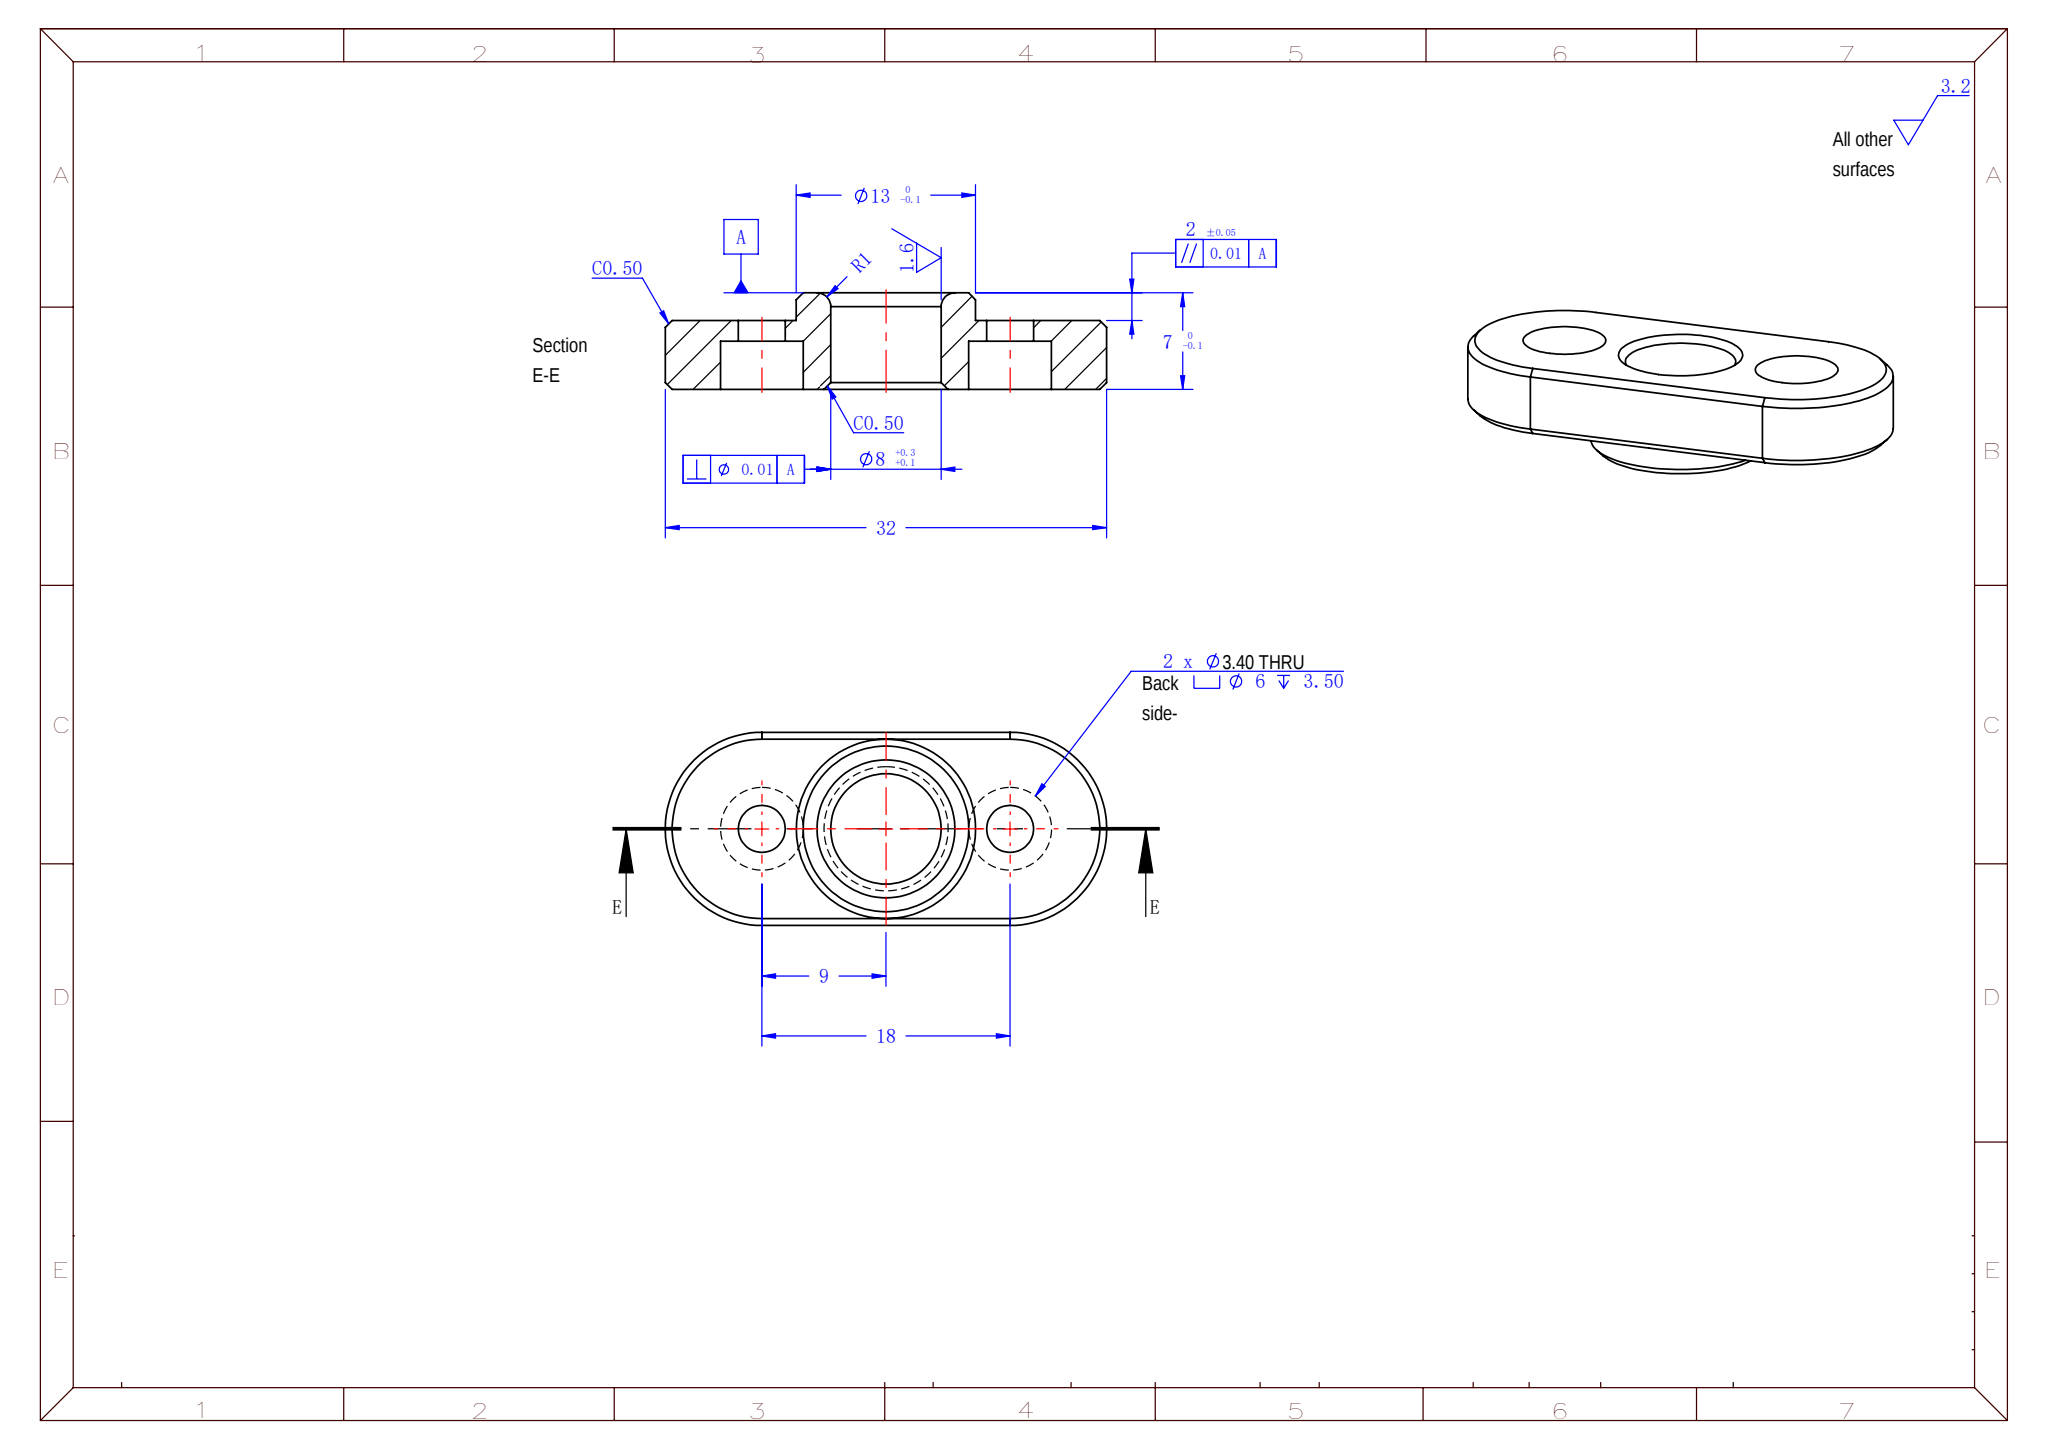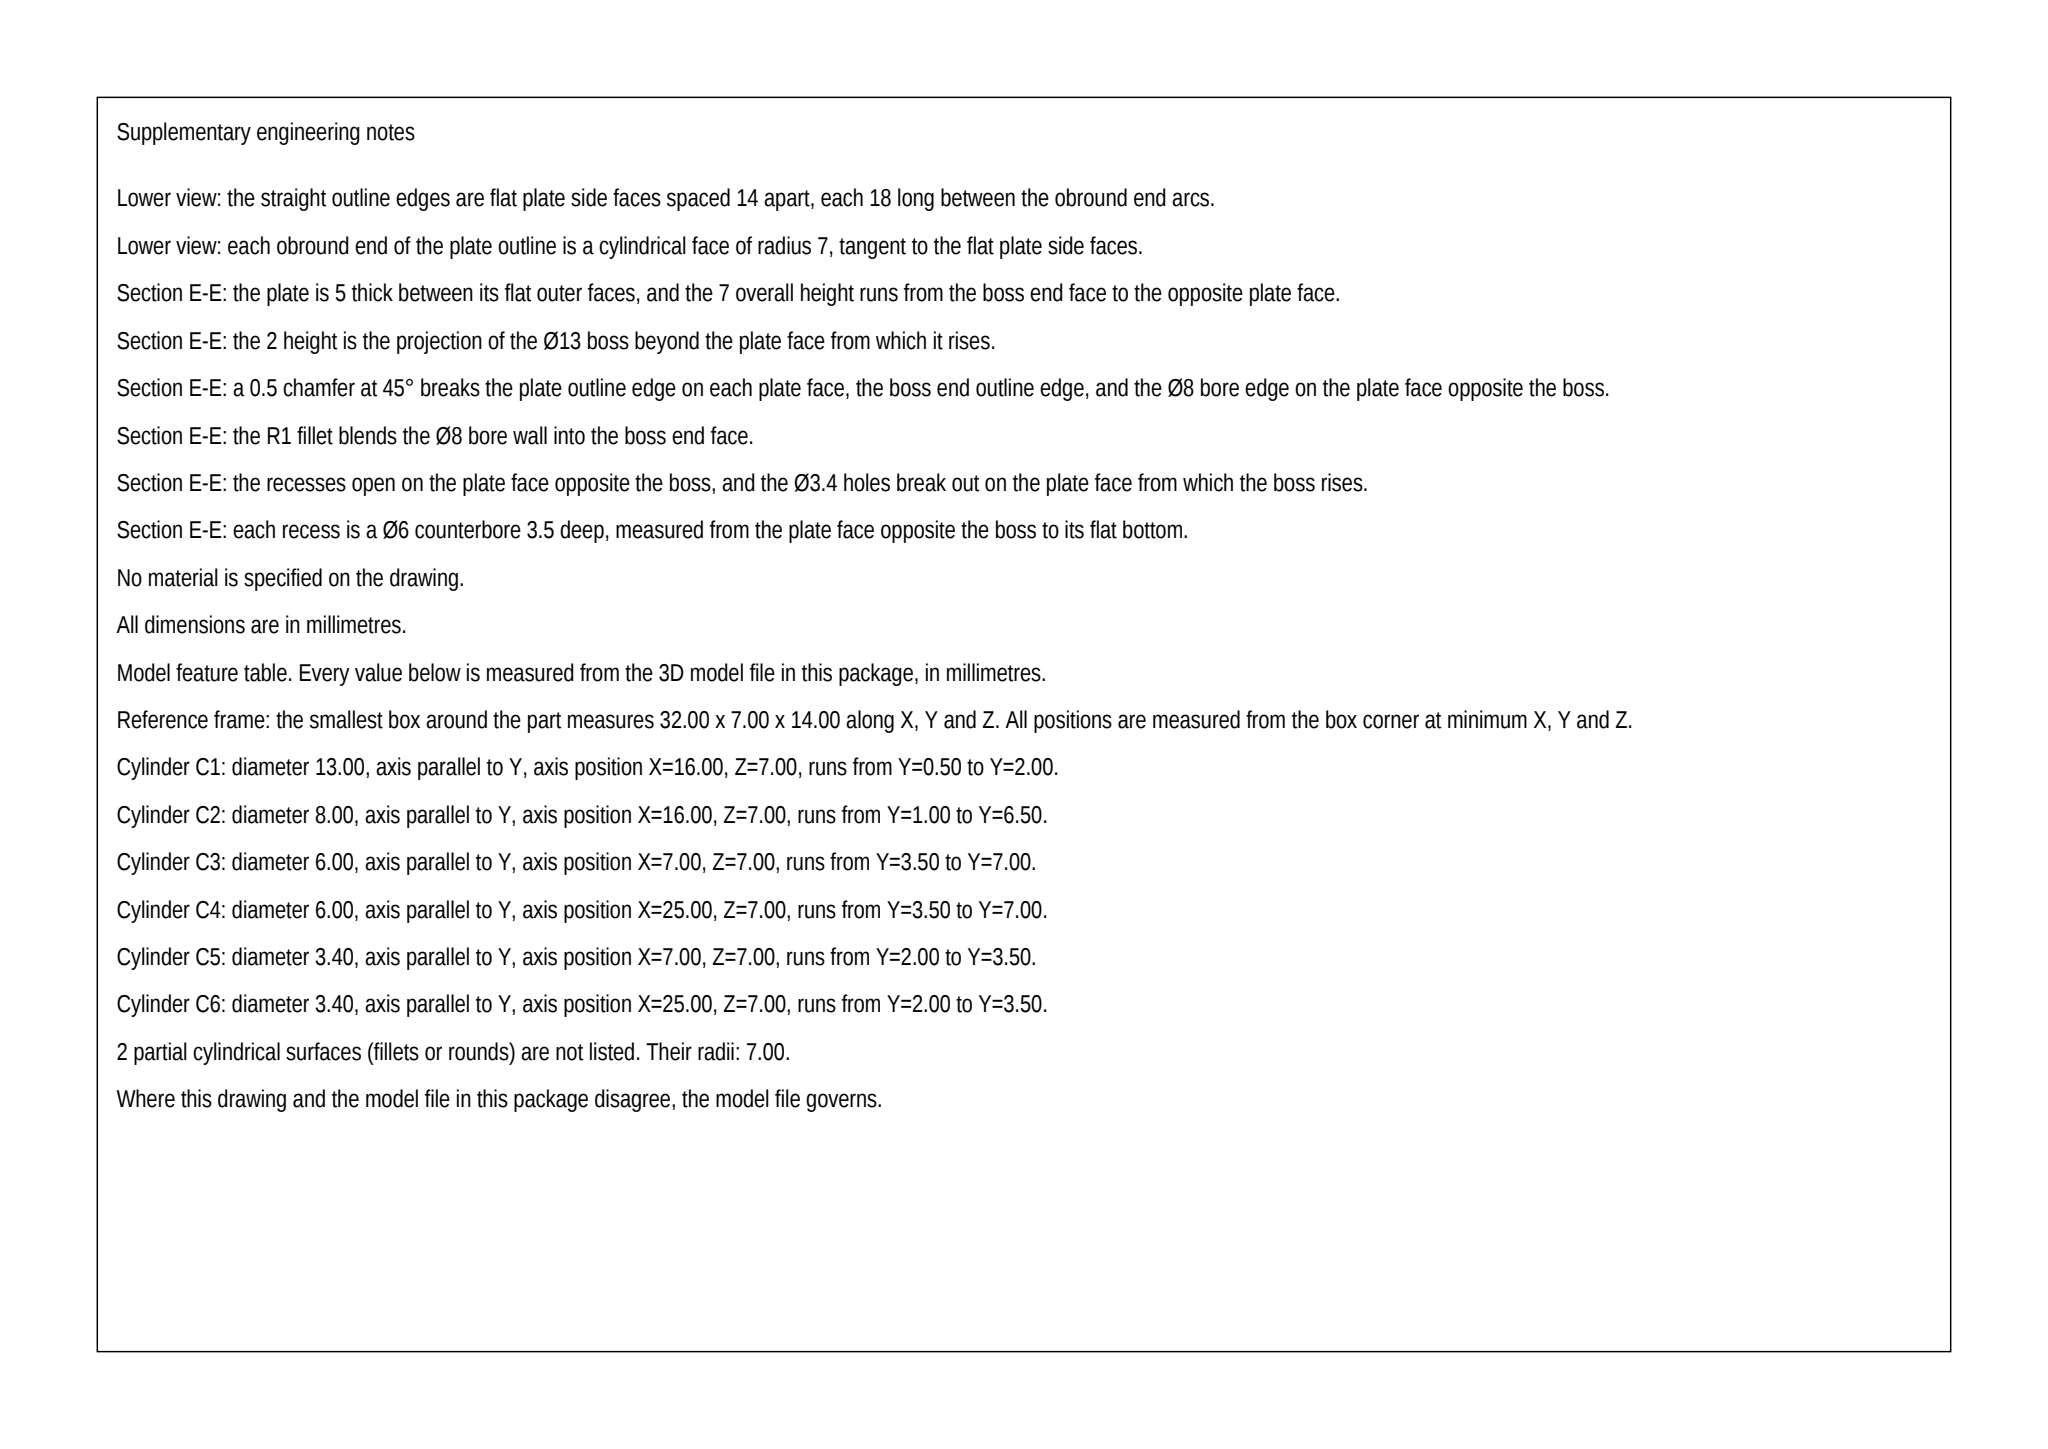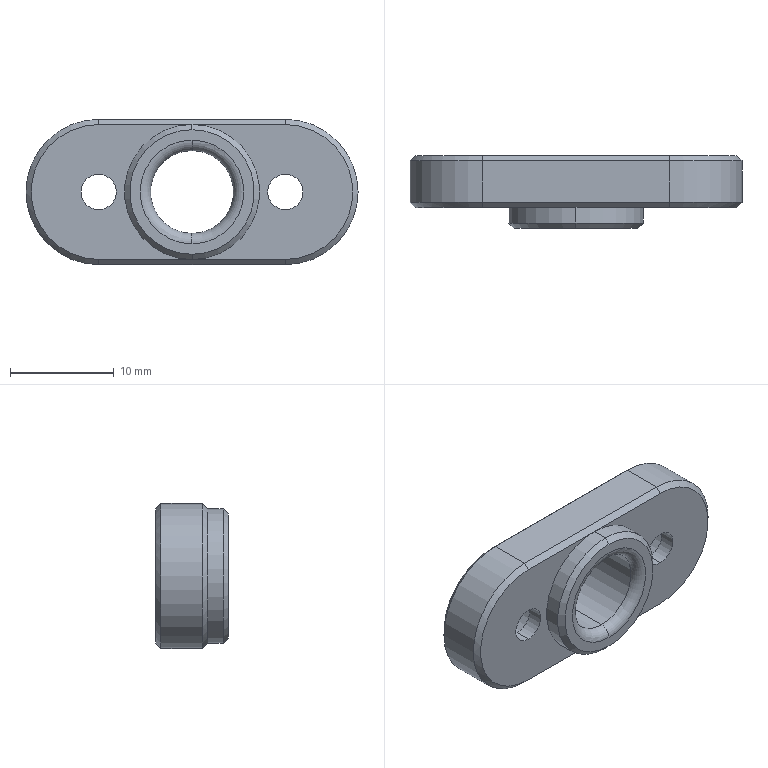Part | SolidWorks | mm | material S45C | 1 solid | 36 faces | box 32 x 7 x 14 mm | volume 1684 mm3 | cylinder 14 | plane 12 | cone 8 | torus 2 | commonest cylinder face diameters 6 x4 3.4 x4 13 x2 8 x2 14 x2
Drawing notes:
2X R7 (Ø14) AT ENDS; OVERALL WIDTH 14 | from the solid: convex arcs dia 14 about y-axis at x=7 & x=25; bbox z extent 14.0